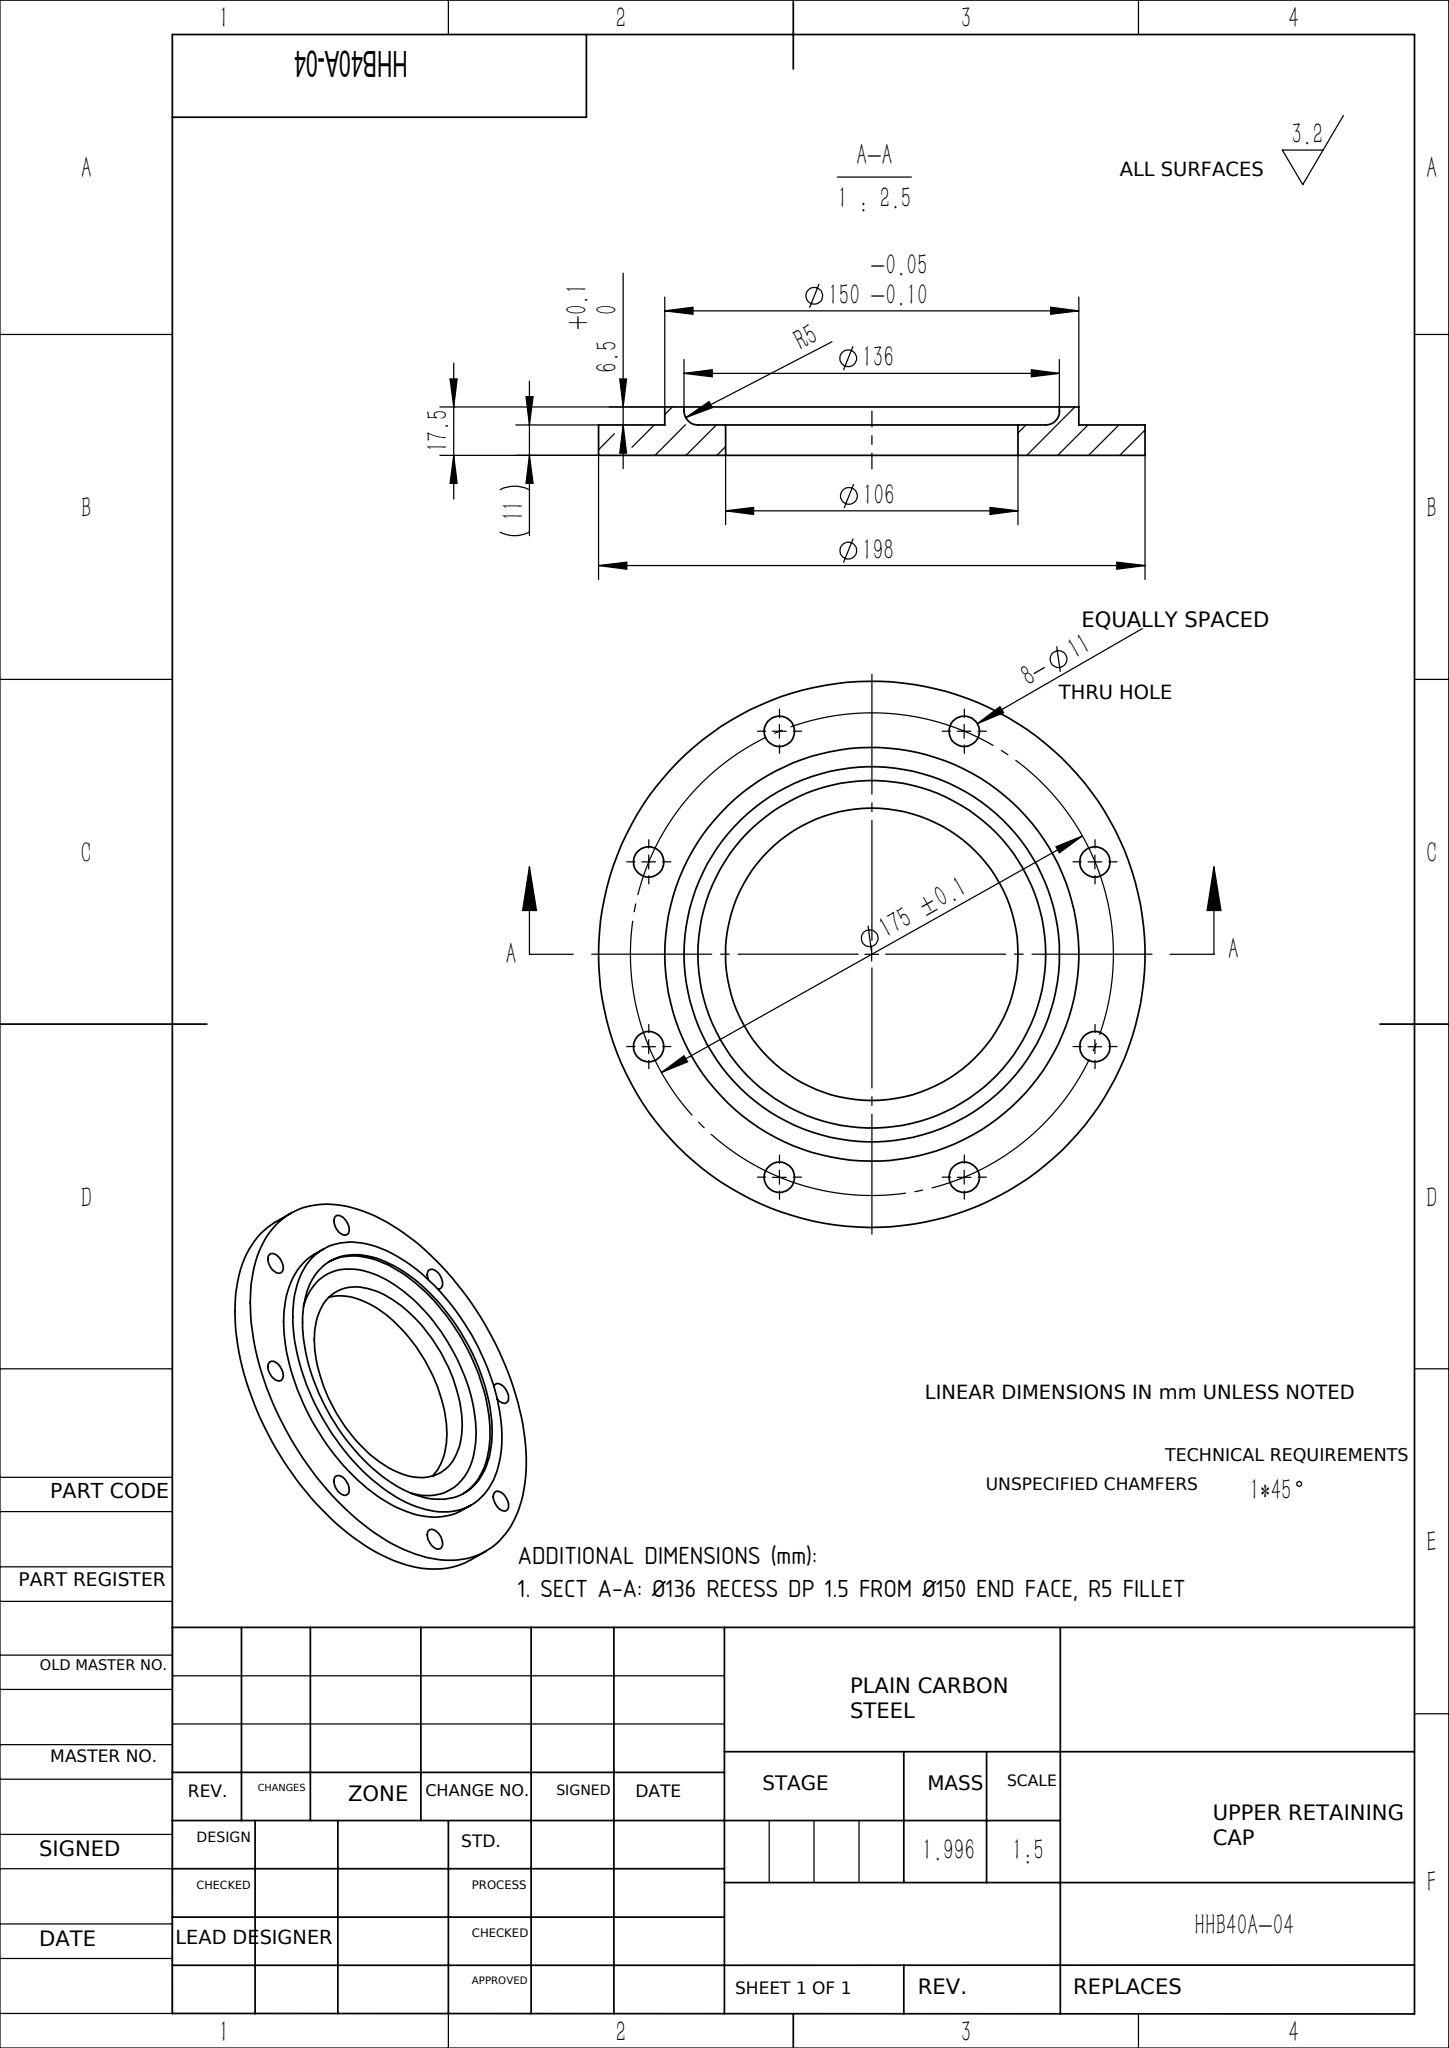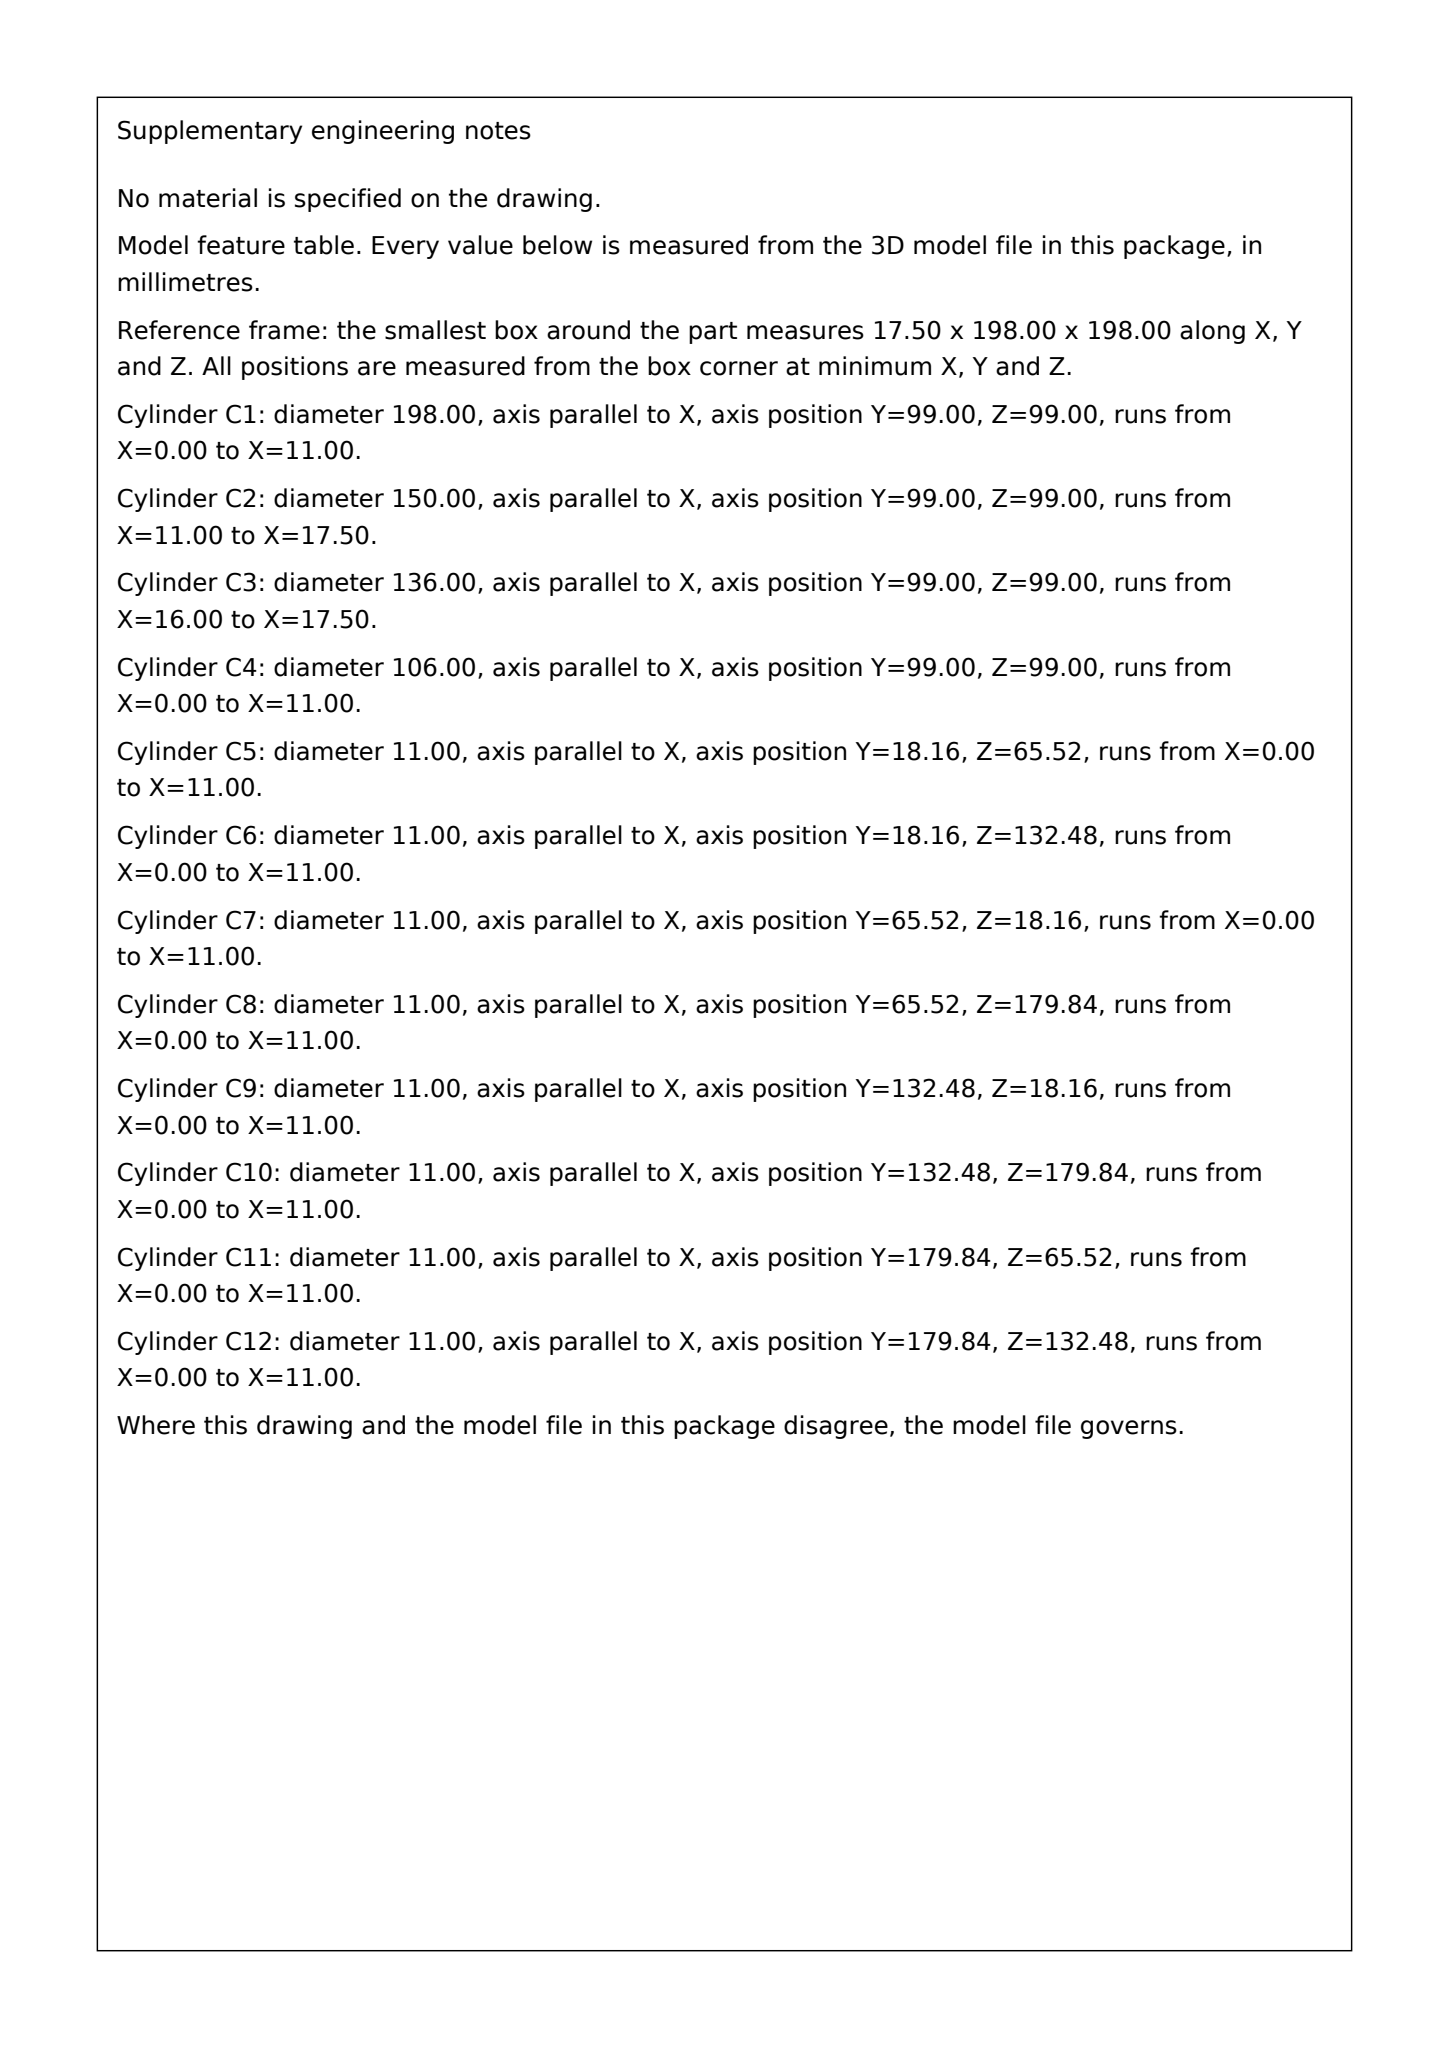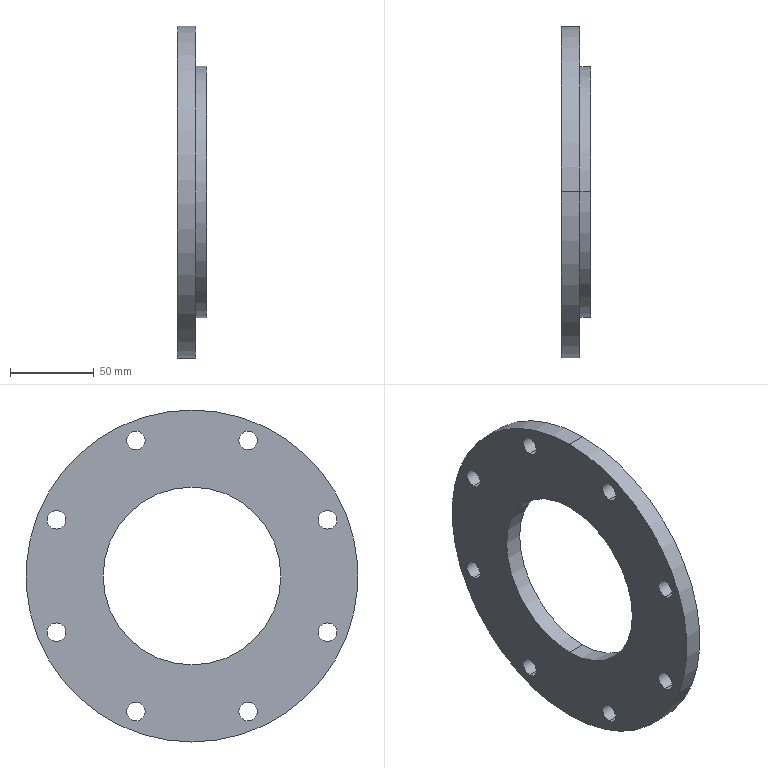Part | SolidWorks | mm | 1 solid | 30 faces | box 17.5 x 198 x 198 mm | volume 255959 mm3 | cylinder 24 | plane 4 | torus 2 | commonest cylinder face diameters 11 x16 136 x2 150 x2 198 x2 106 x2
build123d program:
from build123d import *

# Parameters (mm, degrees)
FILLET1_R          = 5
SKETCH2_R          = 5.5
CUT_EXTRUDE2_DEPTH = 142.097


with BuildPart() as part:
    # Sketch1 → Revolve1 (revolve)
    with BuildSketch(Plane.XY, mode=Mode.PRIVATE) as revolve1_sk:
        Polygon((0, 53), (0, 99), (11, 99), (11, 75), (17.5, 75), (17.5, 68), (11, 68), (11, 53), align=None)
    revolve(revolve1_sk.sketch.rotate(Axis((0, 0, 0), (1, 0, 0)), 90), axis=Axis((0, 0, 0), (1, 0, 0)))

    # Fillet1
    fillet1_edges = [part.edges().sort_by_distance(p)[0] for p in [
        (11, 0, -68),
    ]]
    fillet(fillet1_edges, radius=FILLET1_R)

    # Sketch2 → Cut-Extrude2 (cut, through all)
    with BuildSketch(Plane(origin=(0, 0, 0), x_dir=(0, 0, -1), z_dir=(1, 0, 0))):
        with Locations(Location((80.839, 33.485, 0), (0, 0, 180))):
            Circle(SKETCH2_R)
        with Locations(Location((80.839, -33.485, 0), (0, 0, 180))):
            Circle(SKETCH2_R)
        with Locations(Location((33.485, -80.839, 0), (0, 0, 180))):
            Circle(SKETCH2_R)
        with Locations(Location((-33.485, -80.839, 0), (0, 0, 180))):
            Circle(SKETCH2_R)
        with Locations(Location((-80.839, -33.485, 0), (0, 0, 180))):
            Circle(SKETCH2_R)
        with Locations(Location((-80.839, 33.485, 0), (0, 0, 180))):
            Circle(SKETCH2_R)
        with Locations(Location((-33.485, 80.839, 0), (0, 0, 180))):
            Circle(SKETCH2_R)
        with Locations(Location((33.485, 80.839, 0), (0, 0, 180))):
            Circle(SKETCH2_R)
    extrude(amount=CUT_EXTRUDE2_DEPTH, mode=Mode.SUBTRACT)


solid = part.part